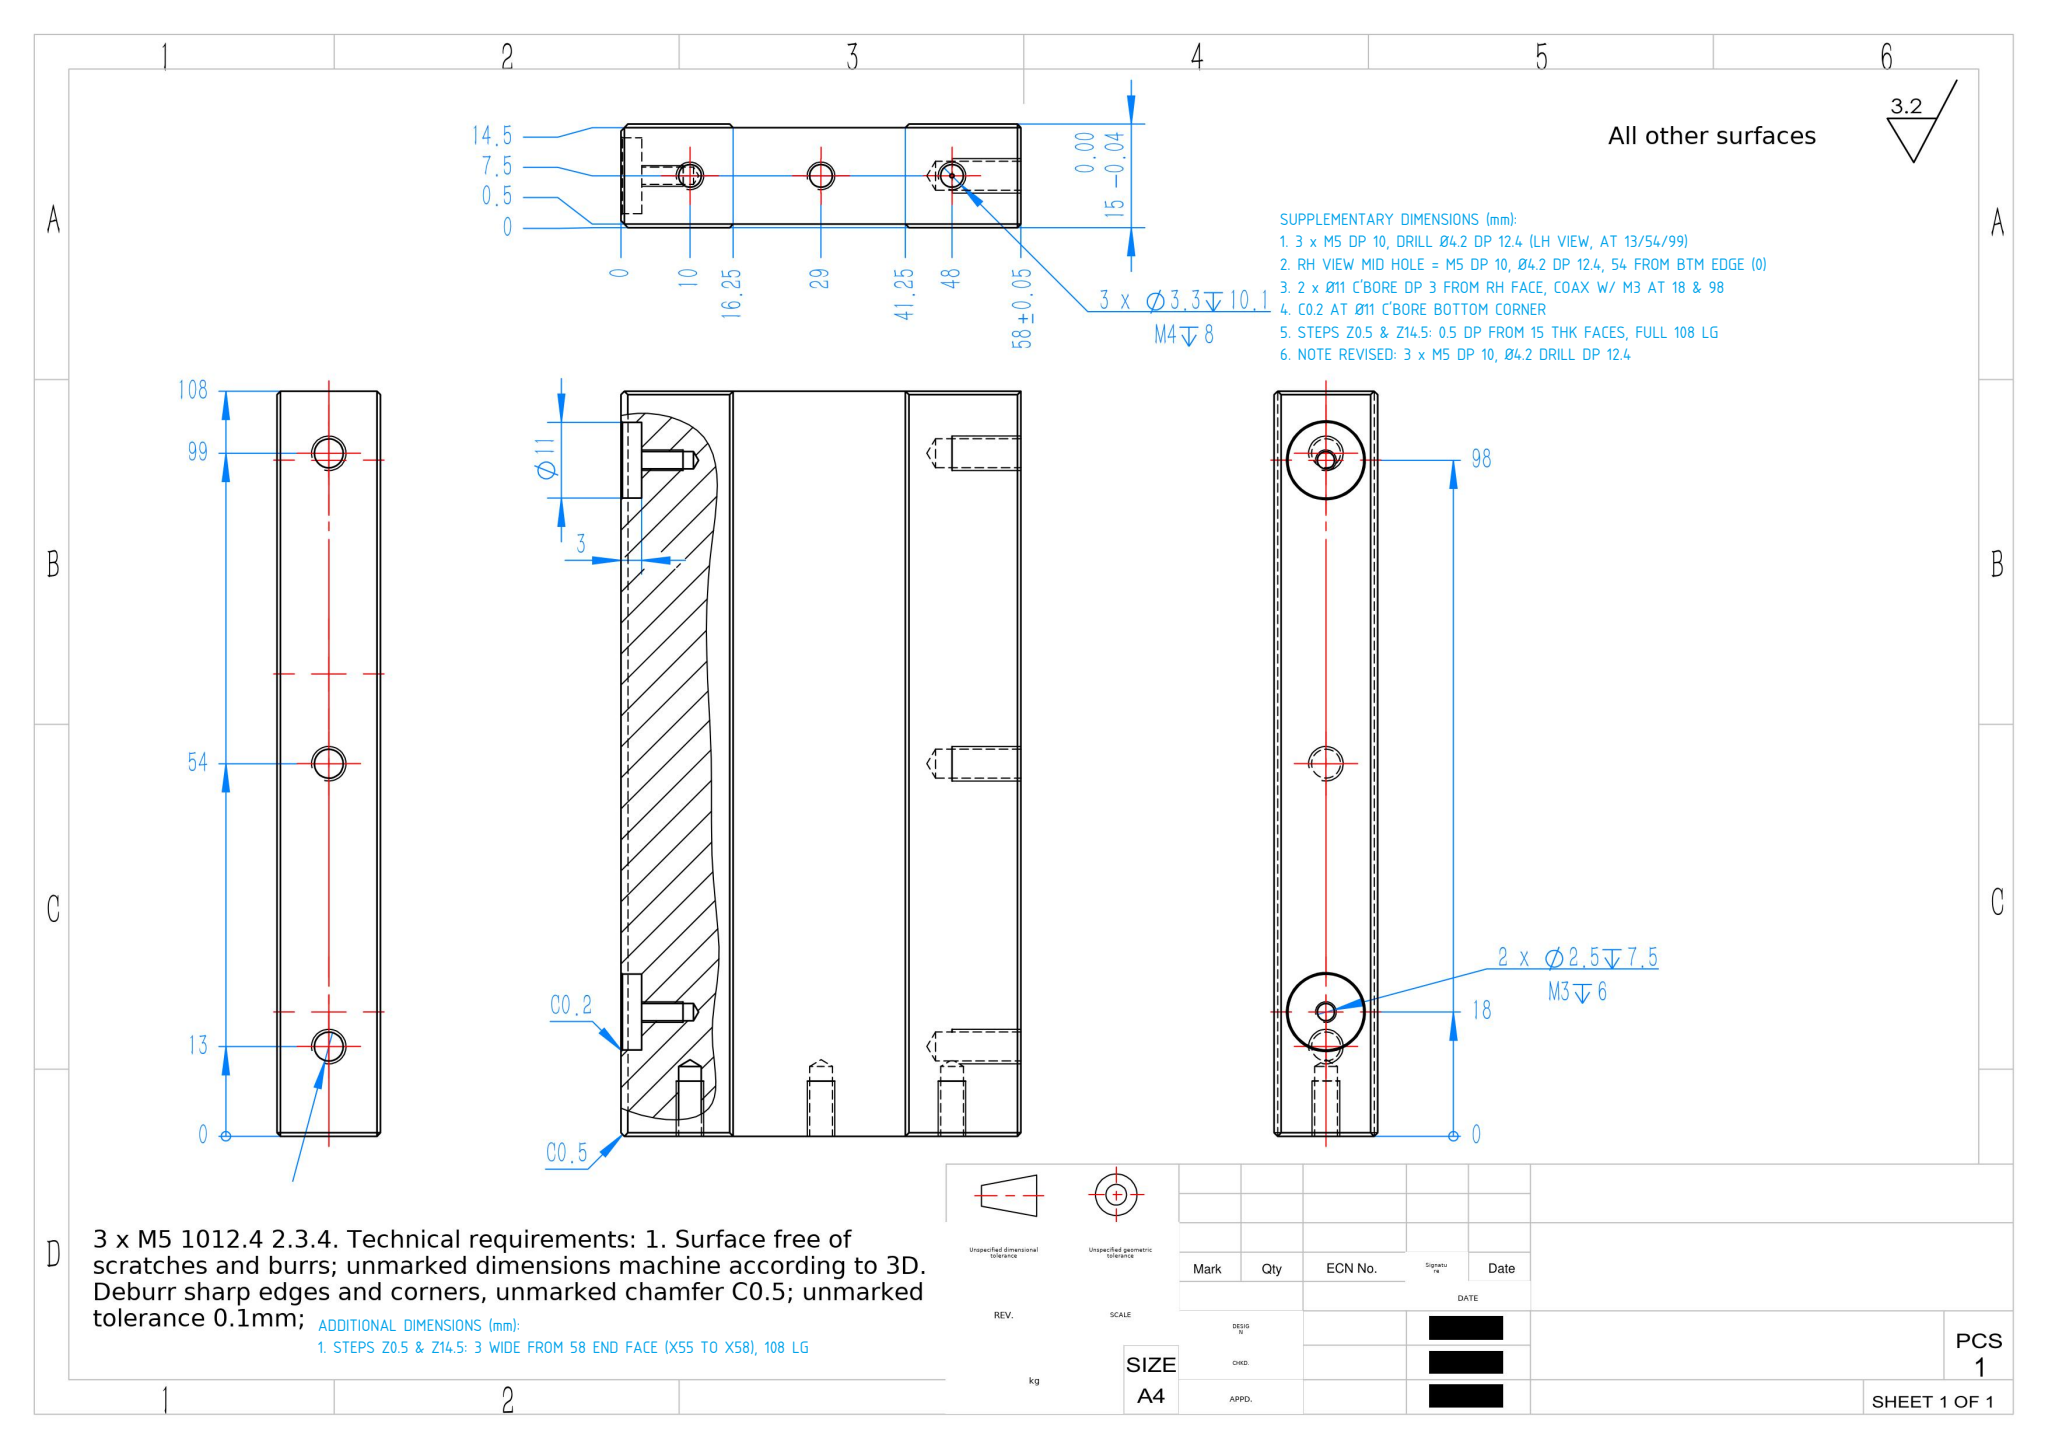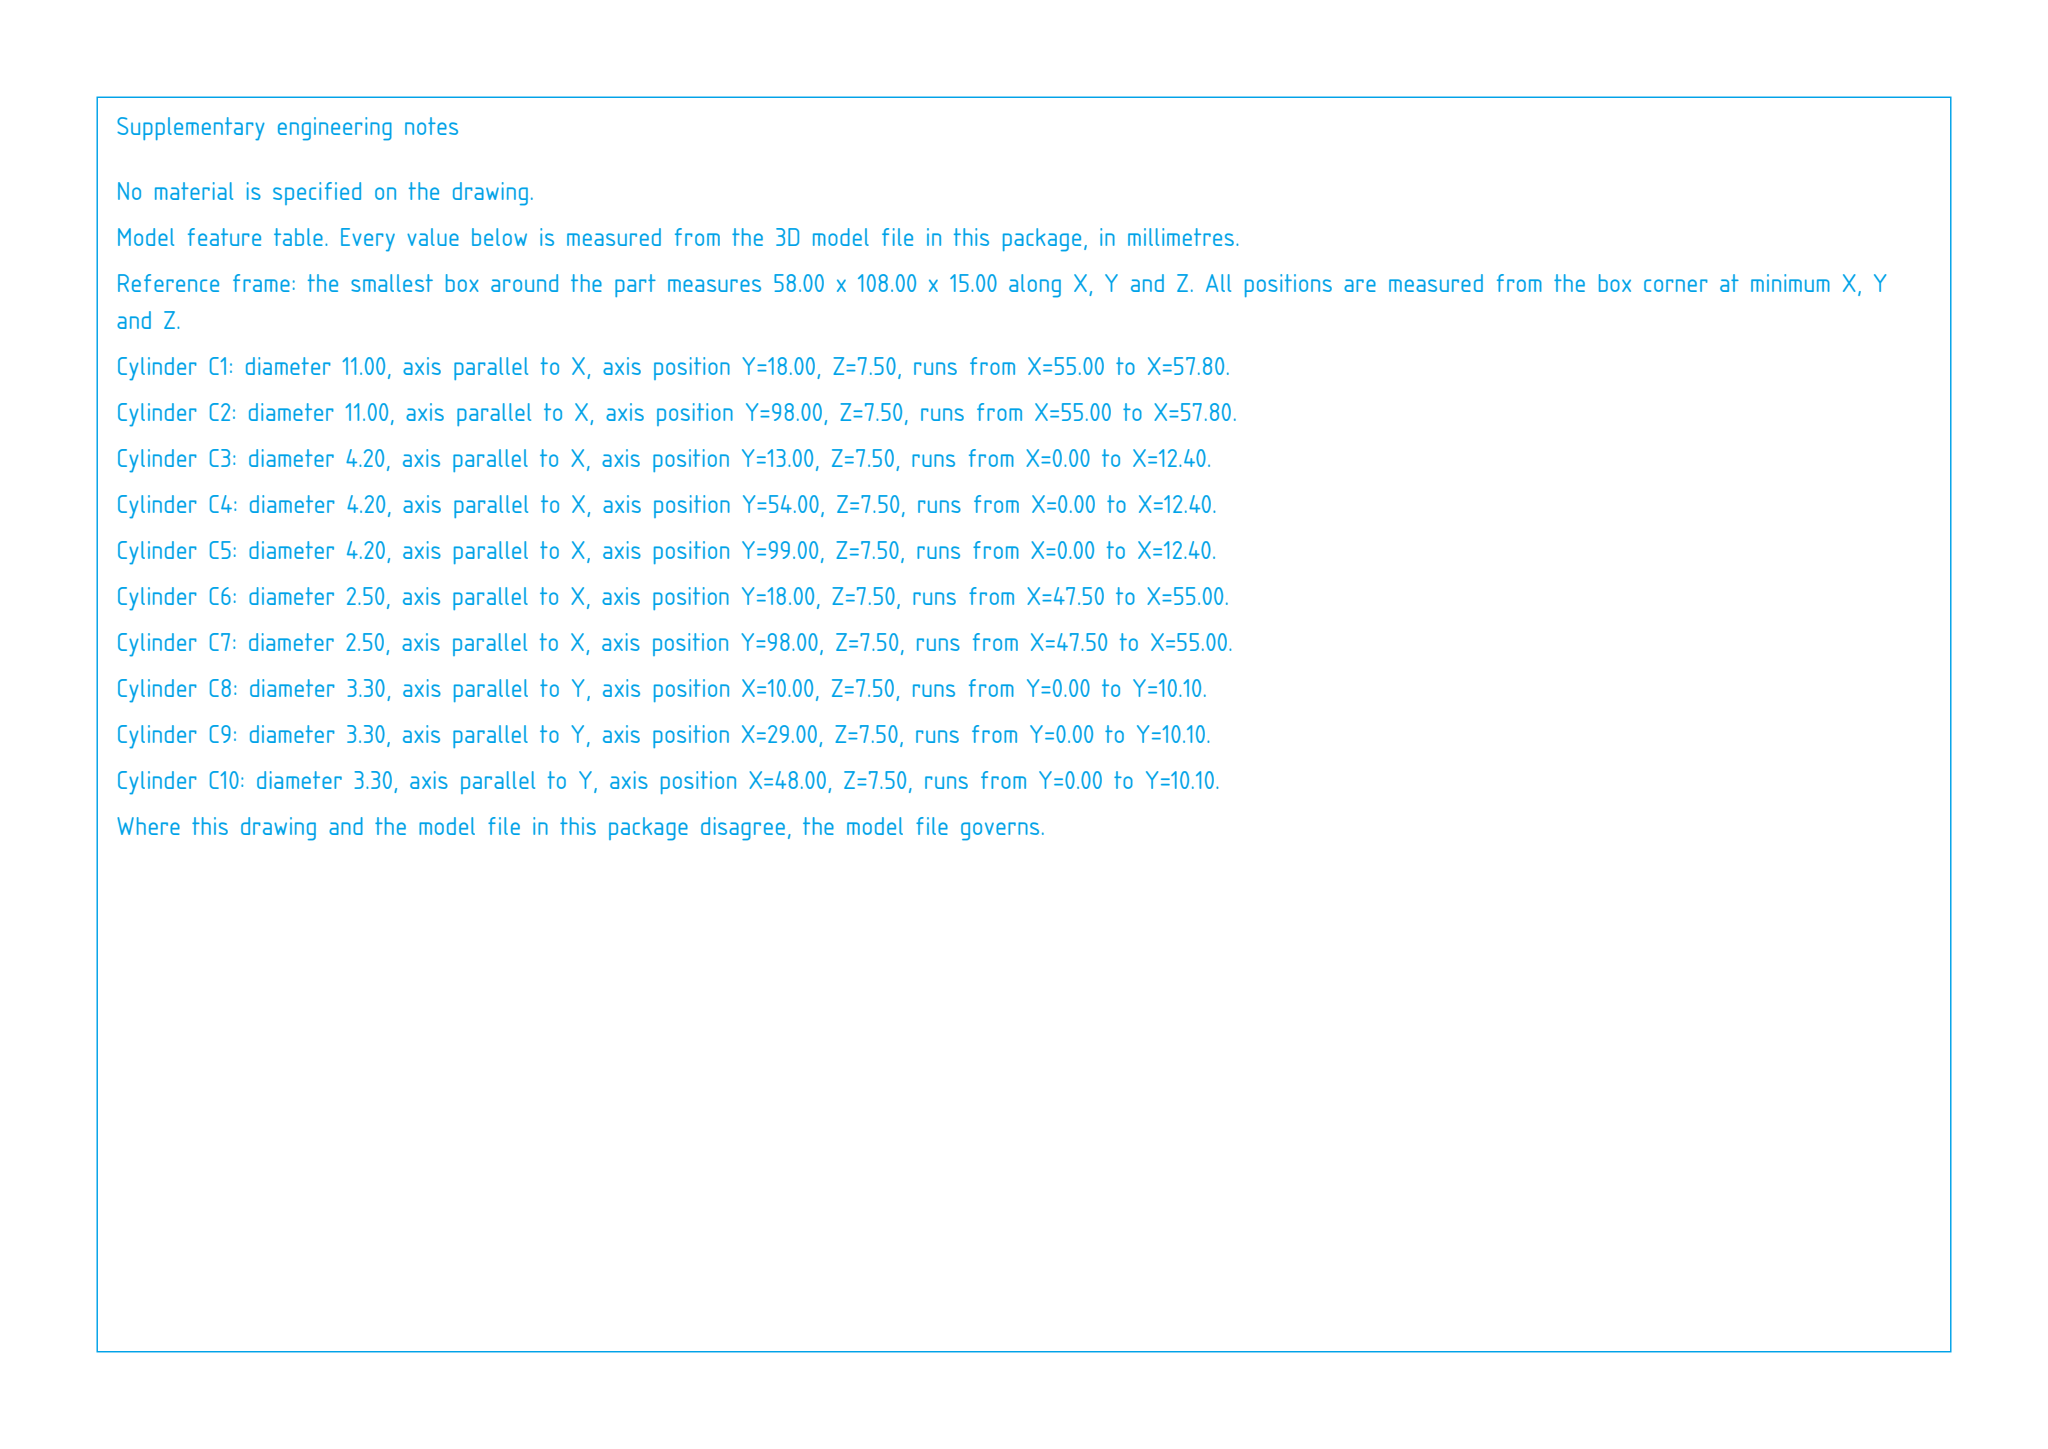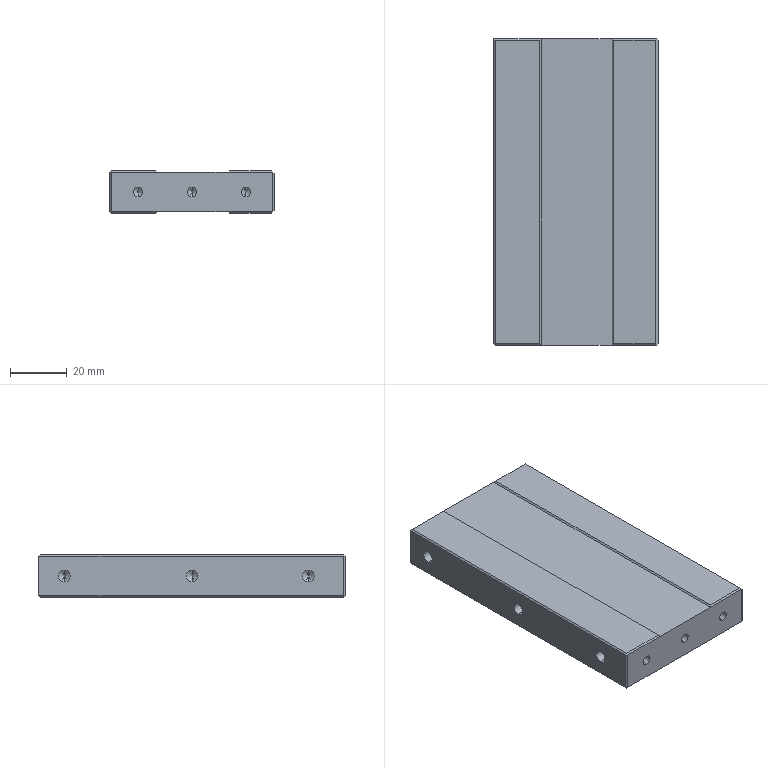Part | SolidWorks | mm | 1 solid | 73 faces | box 58 x 108 x 15 mm | volume 89602 mm3 | plane 33 | cone 20 | cylinder 20 | commonest cylinder face diameters 3.3 x6 4.2 x6 2.5 x4 11 x4